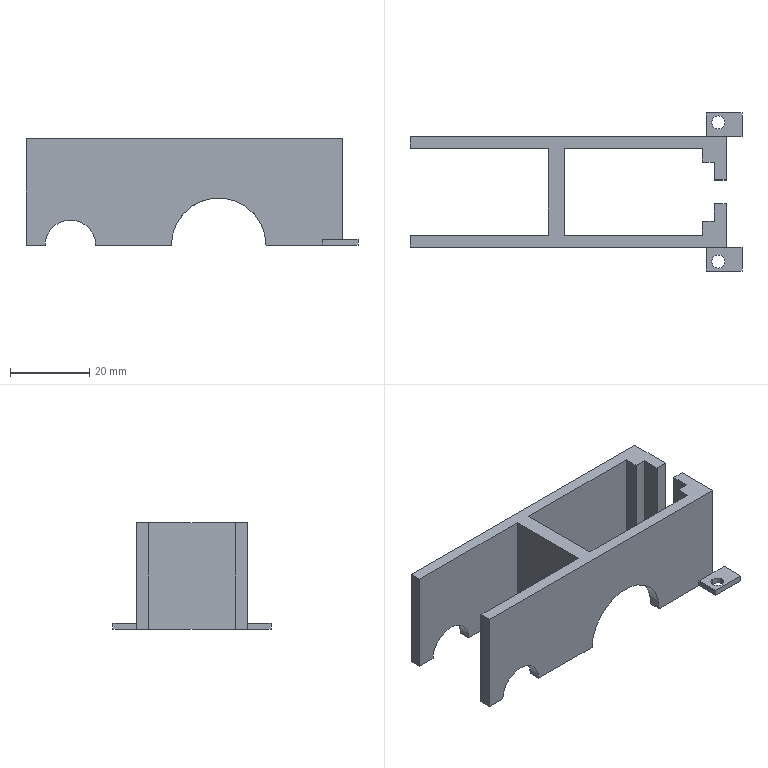Component | SolidWorks | Stabilizer-1 | 1 solid | 45 faces | box 84 x 40 x 27 mm | volume 15357 mm3 | plane 36 | cylinder 9 | commonest cylinder face diameters 12.8 x4 3.3 x4 24 x1
build123d program:
from build123d import *

# Parameters (mm, degrees)
BOSS_EXTRUDE1_DEPTH     = 27
SKETCH2_R               = 12
CUT_EXTRUDE1_DEPTH      = 37
SKETCH3_W               = 6
SKETCH3_H               = 9
SKETCH3_R               = 1.65
BOSS_EXTRUDE2_DEPTH     = 1.5
SKETCH4_W               = 3
SKETCH4_H               = 27
BOSS_EXTRUDE3_DEPTH     = 35
CUT_EXTRUDE2_DEPTH      = 30
CUT_EXTRUDE2_DEPTH_BACK = 10
SKETCH6_R               = 6.4


with BuildPart() as part:
    # Sketch1 → Boss-Extrude1 (new body)
    with BuildSketch(Plane.XY):
        Polygon((11, 42), (11, 45), (0, 45), (0, 0), (28, 0), (28, 45), (17, 45), (17, 42), (21.5, 42), (21.5, 39), (25, 39), (25, 4), (3, 4), (3, 39), (6.5, 39), (6.5, 42), align=None)
    extrude(amount=BOSS_EXTRUDE1_DEPTH)

    # Sketch2 → Cut-Extrude1 (cut)
    with BuildSketch(Plane.ZY):
        with Locations((0, 13.75)):
            Circle(SKETCH2_R)
    extrude(amount=-CUT_EXTRUDE1_DEPTH, mode=Mode.SUBTRACT)

    # Sketch3 → Boss-Extrude2 (add)
    # profile 1 of 2: a face of its own
    with BuildSketch(Plane(origin=(0, 0, 0), x_dir=(-1, 0, 0), z_dir=(0, 0, -1))):
        with Locations((3, 44.5)):
            Rectangle(SKETCH3_W, SKETCH3_H)
        with Locations((3.6, 43)):
            Circle(SKETCH3_R, mode=Mode.SUBTRACT)
    # profile 2 of 2: a face of its own
    with BuildSketch(Plane(origin=(0, 0, 0), x_dir=(-1, 0, 0), z_dir=(0, 0, -1))):
        with Locations((-31, 44.5)):
            Rectangle(SKETCH3_W, SKETCH3_H)
        with Locations(Location((-31.6, 43, 0), (0, 0, 180))):
            Circle(SKETCH3_R, mode=Mode.SUBTRACT)
    extrude(amount=-BOSS_EXTRUDE2_DEPTH)

    # Sketch4 → Boss-Extrude3 (add)
    with BuildSketch(Plane.XZ):
        with Locations((1.5, 13.5)):
            Rectangle(SKETCH4_W, SKETCH4_H)
        with Locations((26.5, 13.5)):
            Rectangle(SKETCH4_W, SKETCH4_H)
    extrude(amount=BOSS_EXTRUDE3_DEPTH)

    # Sketch6 → Cut-Extrude2 (cut, two sides: drawn at the far end of the back side and taken through both)
    with BuildSketch(Plane(origin=(3, 0, 0), x_dir=(0, 0, -1), z_dir=(1, 0, 0)).offset(-CUT_EXTRUDE2_DEPTH_BACK)):
        with Locations((0, -23.761)):
            Circle(SKETCH6_R)
    extrude(amount=CUT_EXTRUDE2_DEPTH + CUT_EXTRUDE2_DEPTH_BACK, mode=Mode.SUBTRACT)


solid = part.part

# Placed as in the assembly
solid = solid.moved(Location((-78.793, 516.247, 900.064), (0, 0, -90)))